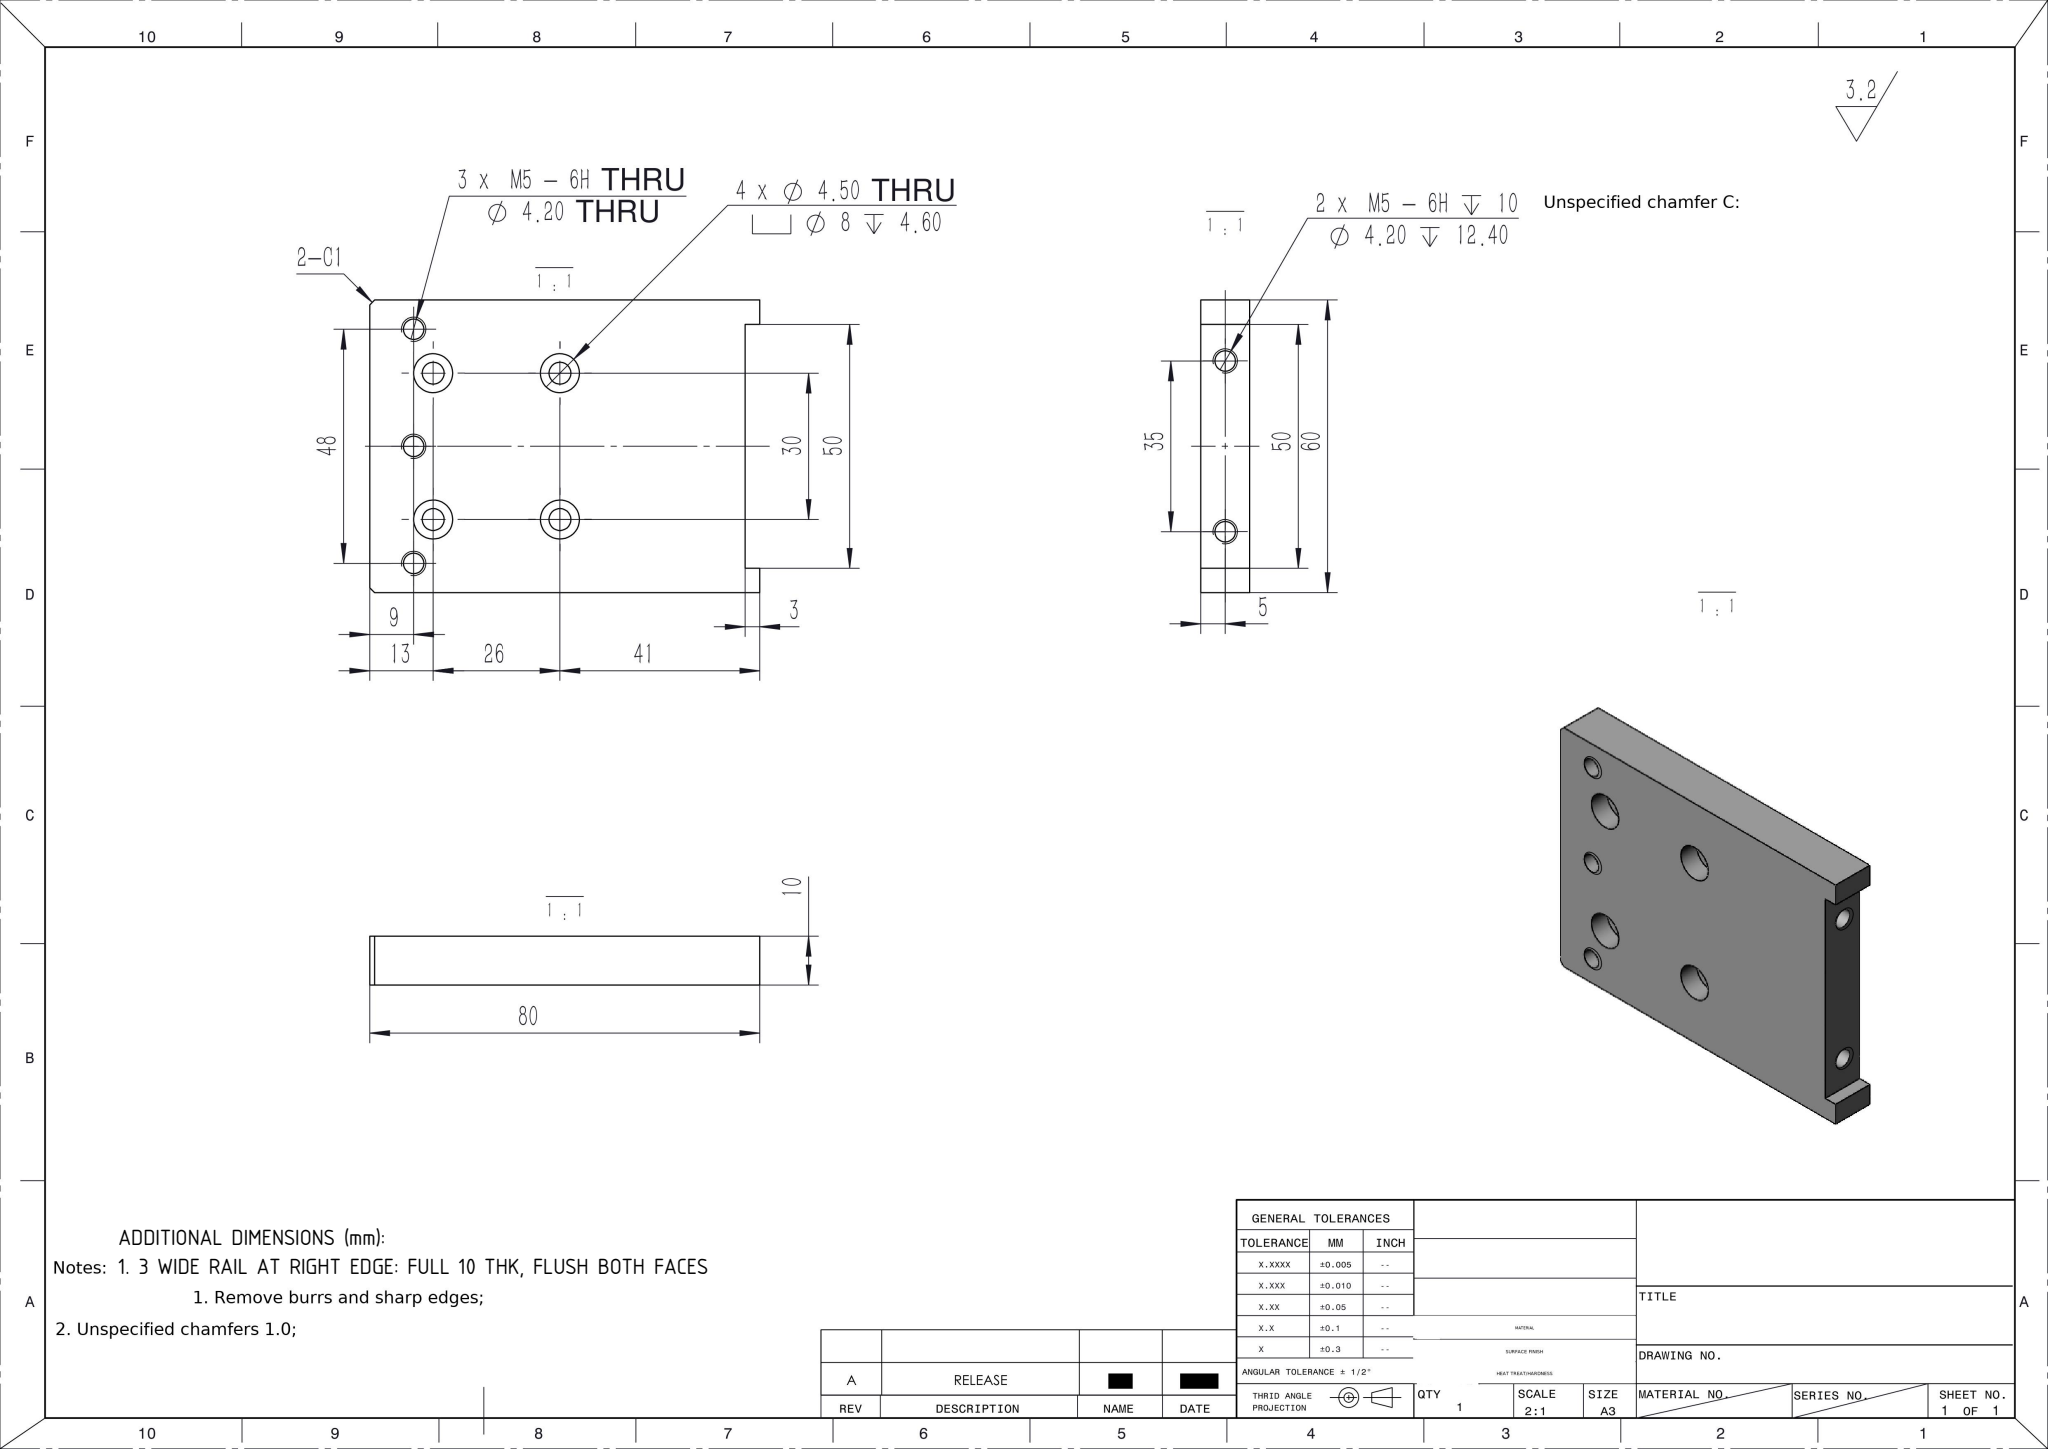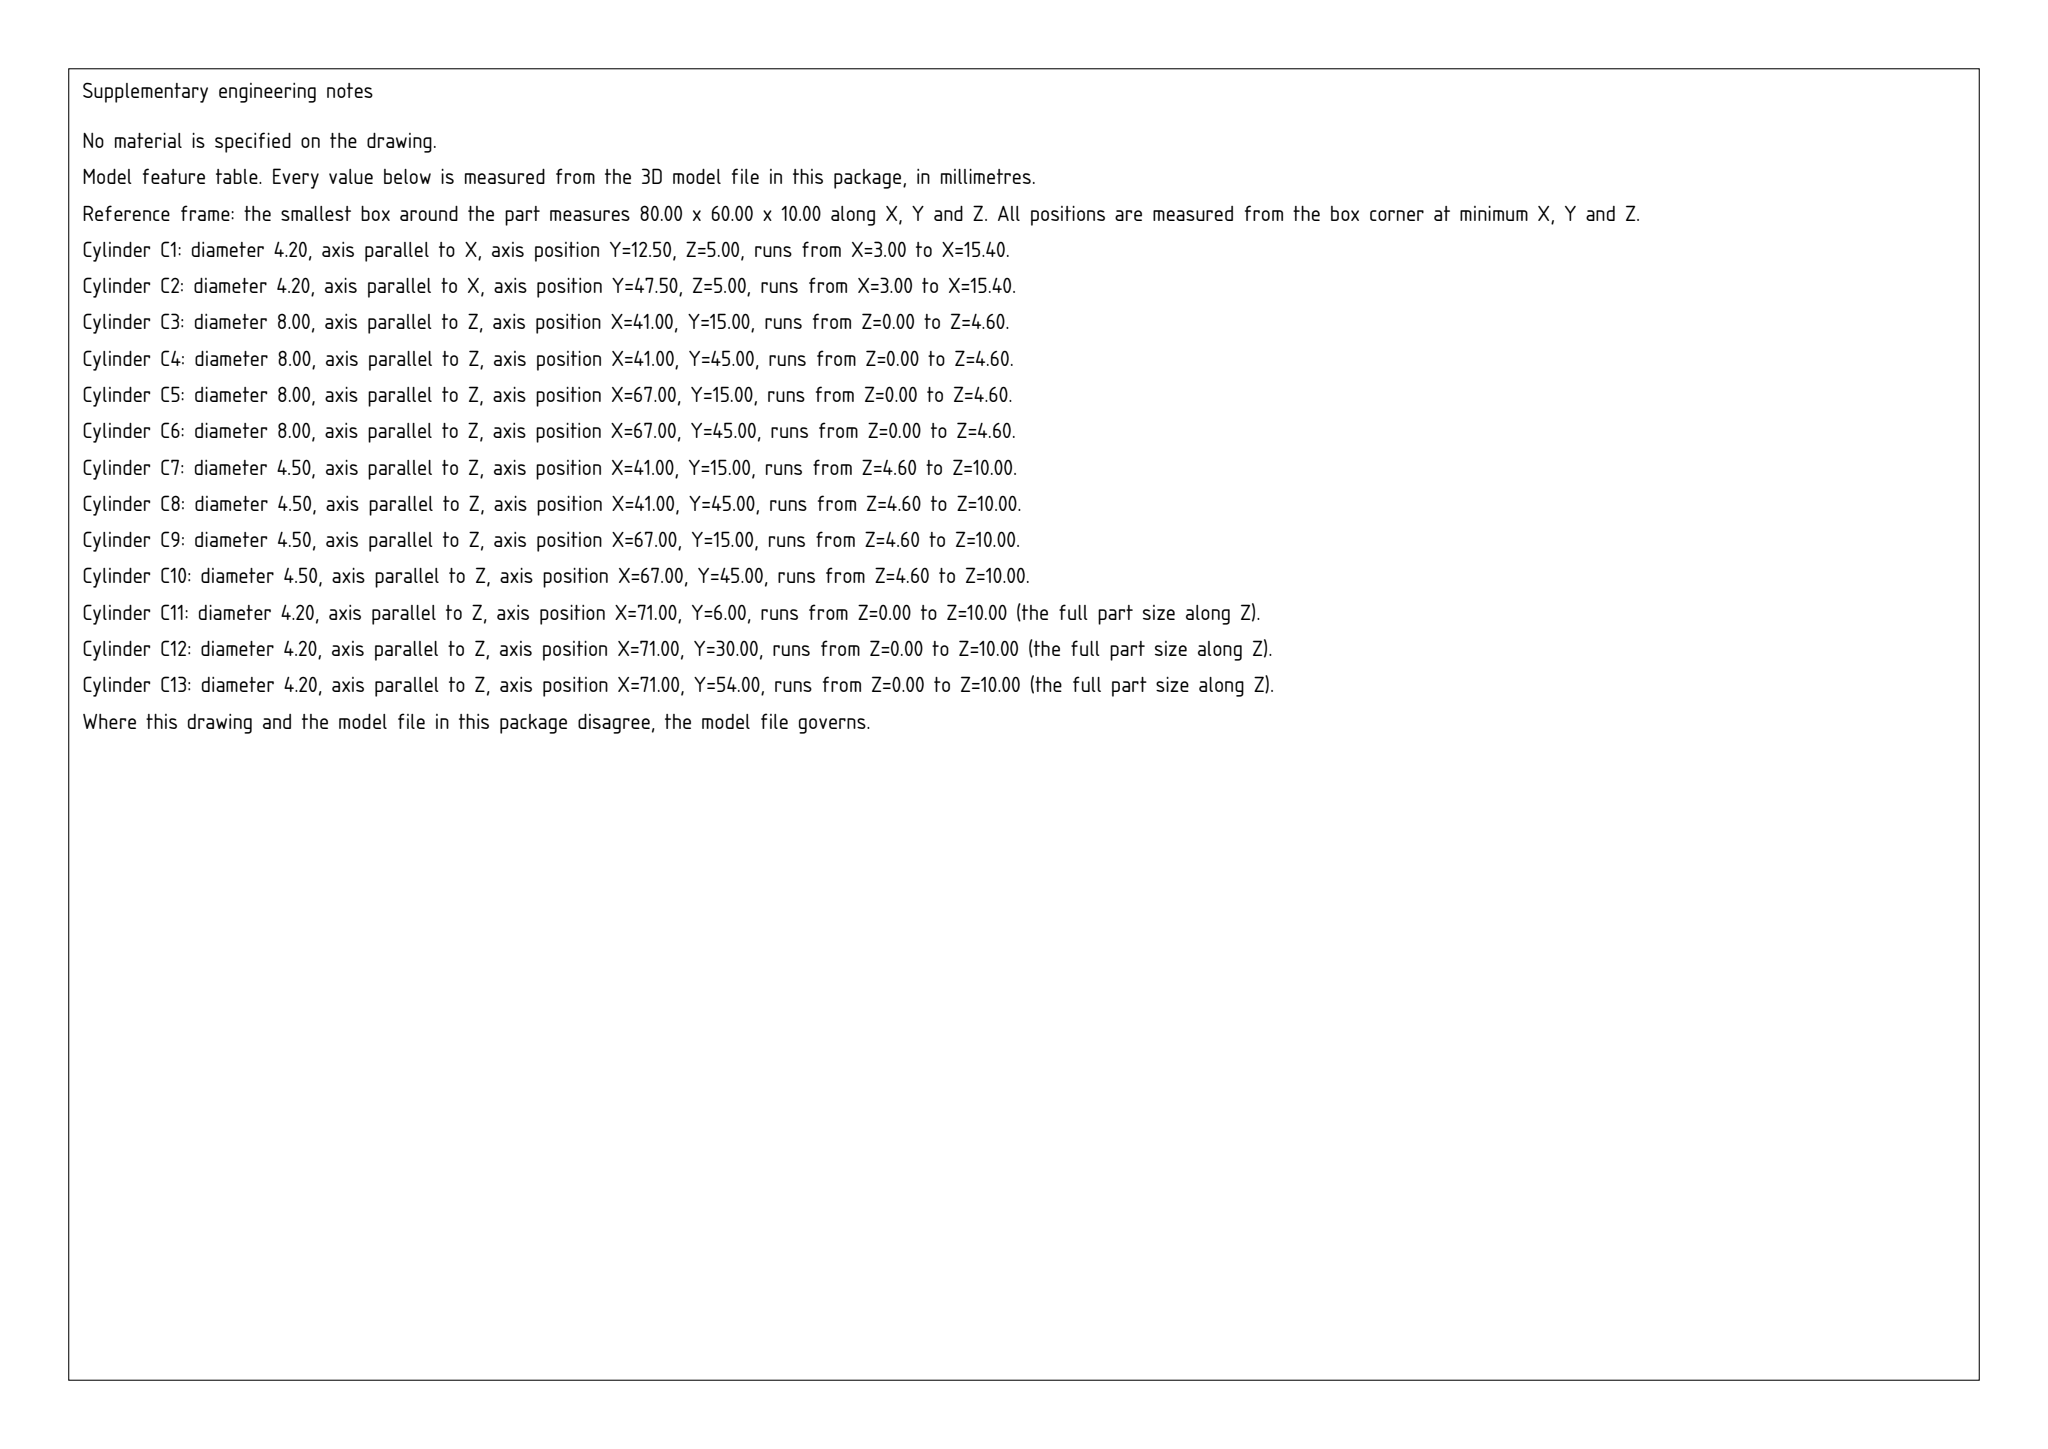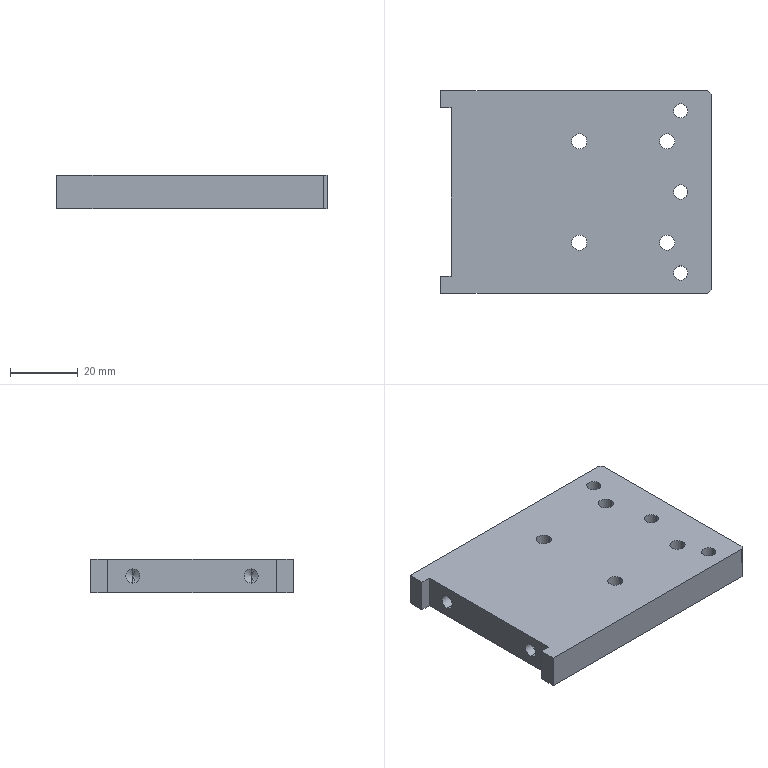Part | SolidWorks | mm | 1 solid | 46 faces | box 80 x 60 x 10 mm | volume 44451 mm3 | cylinder 26 | plane 16 | cone 4 | commonest cylinder face diameters 4.2 x10 8 x8 4.5 x8
build123d program:
from build123d import *

# Parameters (mm, degrees)
SKETCH1_W                                         = 80
SKETCH1_H                                         = 60
BOSS_EXTRUDE1_DEPTH                               = 10
HOLE_SIZE_ACCORDING_TO_HEXAGON_SOCKET_D           = 4.5
HOLE_SIZE_ACCORDING_TO_HEXAGON_SOCKET_CBORE_D     = 8
HOLE_SIZE_ACCORDING_TO_HEXAGON_SOCKET_CBORE_DEPTH = 4.6
M5_TAPPED_HOLE1_D                                 = 4.2
SKETCH10_W                                        = 6
SKETCH10_H                                        = 50
CUT_EXTRUDE1_DEPTH                                = 51.99
M5_TAPPED_HOLE2_D                                 = 4.2
M5_TAPPED_HOLE2_DEPTH                             = 12.4
M5_TAPPED_HOLE2_TIP                               = 1.262
CHAMFER1_SIZE                                     = 1


with BuildPart() as part:
    # Sketch1 → Boss-Extrude1 (new body)
    with BuildSketch(Plane.XY):
        Rectangle(SKETCH1_W, SKETCH1_H)
    extrude(amount=BOSS_EXTRUDE1_DEPTH)

    # Hole Size _ according to_ Hexagon Socket (through all)
    with Locations(Plane(origin=(0, 0, 0), x_dir=(-1, 0, 0), z_dir=(0, 0, -1))):
        with Locations((-27, -15), (-1, -15), (-1, 15), (-27, 15)):
            CounterBoreHole(HOLE_SIZE_ACCORDING_TO_HEXAGON_SOCKET_D / 2, HOLE_SIZE_ACCORDING_TO_HEXAGON_SOCKET_CBORE_D / 2, HOLE_SIZE_ACCORDING_TO_HEXAGON_SOCKET_CBORE_DEPTH)

    # M5 Tapped Hole1 (through all)
    with Locations(Plane(origin=(0, 0, 0), x_dir=(-1, 0, 0), z_dir=(0, 0, -1))):
        with Locations((-31, 24), (-31, 0), (-31, -24)):
            Hole(M5_TAPPED_HOLE1_D / 2)

    # Sketch10 → Cut-Extrude1 (cut, through all)
    with BuildSketch(Plane(origin=(0, 0, 0), x_dir=(-1, 0, 0), z_dir=(0, 0, -1))):
        with Locations((40, 0)):
            Rectangle(SKETCH10_W, SKETCH10_H)
    extrude(amount=-CUT_EXTRUDE1_DEPTH, mode=Mode.SUBTRACT)

    # M5 Tapped Hole2
    with Locations(Plane.ZY.offset(37)):
        with Locations((5, 17.5), (5, -17.5)):
            Hole(M5_TAPPED_HOLE2_D / 2, depth=M5_TAPPED_HOLE2_DEPTH)
            with Locations((0, 0, -(M5_TAPPED_HOLE2_DEPTH + M5_TAPPED_HOLE2_TIP / 2))):  # 118° drill point
                Cone(0, M5_TAPPED_HOLE2_D / 2, M5_TAPPED_HOLE2_TIP, mode=Mode.SUBTRACT)

    # Chamfer1
    chamfer1_edges = [part.edges().sort_by_distance(p)[0] for p in [
        (40, -30, 5),
        (40, 30, 5),
    ]]
    chamfer(chamfer1_edges, length=CHAMFER1_SIZE)


solid = part.part